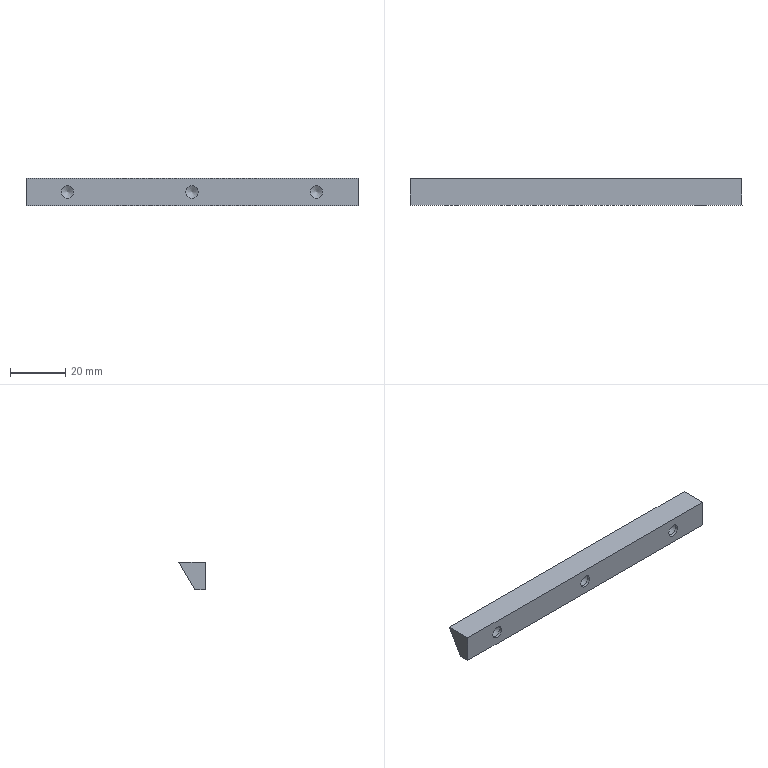Component | NX | SLIDE_GIB_2 | 1 solid | 12 faces | box 120 x 9.5 x 10 mm | volume 7867 mm3 | plane 6 | cone 3 | cylinder 3 | commonest cylinder face diameters 4.5 x3
STEP:
#1=CARTESIAN_POINT('',(0.,0.,0.));
#2=DIRECTION('',(0.,0.,1.));
#3=DIRECTION('',(1.,0.,0.));
#4=AXIS2_PLACEMENT_3D('',#1,#2,#3);
#5=CARTESIAN_POINT('',(-59.8,-54.082,73.));
#6=VERTEX_POINT('',#5);
#7=CARTESIAN_POINT('',(-59.8,-63.582,73.));
#8=VERTEX_POINT('',#7);
#9=CARTESIAN_POINT('',(-59.8,-54.082,73.));
#10=DIRECTION('',(0.,-1.,0.));
#11=VECTOR('',#10,1.);
#12=LINE('',#9,#11);
#13=CARTESIAN_POINT('',(60.2,-54.082,73.));
#14=DIRECTION('',(0.,-0.,-1.));
#15=DIRECTION('',(0.,-1.,0.));
#16=AXIS2_PLACEMENT_3D('',#13,#14,#15);
#17=PLANE('',#16);
#18=CARTESIAN_POINT('',(-0.,120.));
#19=DIRECTION('',(1.,-0.));
#20=VECTOR('',#19,1.);
#21=LINE('',#18,#20);
#22=(GEOMETRIC_REPRESENTATION_CONTEXT(2)PARAMETRIC_REPRESENTATION_CONTEXT()REPRESENTATION_CONTEXT('',''));
#23=DEFINITIONAL_REPRESENTATION('',(#21),#22);
#24=PCURVE('',#17,#23);
#25=CARTESIAN_POINT('',(-59.8,-63.582,68.));
#26=DIRECTION('',(1.,0.,0.));
#27=DIRECTION('',(0.,-1.,0.));
#28=AXIS2_PLACEMENT_3D('',#25,#26,#27);
#29=PLANE('',#28);
#30=CARTESIAN_POINT('',(-9.5,-5.));
#31=DIRECTION('',(1.,-0.));
#32=VECTOR('',#31,1.);
#33=LINE('',#30,#32);
#34=(GEOMETRIC_REPRESENTATION_CONTEXT(2)PARAMETRIC_REPRESENTATION_CONTEXT()REPRESENTATION_CONTEXT('',''));
#35=DEFINITIONAL_REPRESENTATION('',(#33),#34);
#36=PCURVE('',#29,#35);
#37=SURFACE_CURVE('',#12,(#24,#36),.PCURVE_S1.);
#38=EDGE_CURVE('',#6,#8,#37,.T.);
#39=ORIENTED_EDGE('',*,*,#38,.T.);
#40=CARTESIAN_POINT('',(60.2,-63.582,73.));
#41=VERTEX_POINT('',#40);
#42=CARTESIAN_POINT('',(60.2,-63.582,73.));
#43=DIRECTION('',(-1.,-0.,0.));
#44=VECTOR('',#43,1.);
#45=LINE('',#42,#44);
#46=CARTESIAN_POINT('',(9.5,0.));
#47=DIRECTION('',(0.,1.));
#48=VECTOR('',#47,1.);
#49=LINE('',#46,#48);
#50=(GEOMETRIC_REPRESENTATION_CONTEXT(2)PARAMETRIC_REPRESENTATION_CONTEXT()REPRESENTATION_CONTEXT('',''));
#51=DEFINITIONAL_REPRESENTATION('',(#49),#50);
#52=PCURVE('',#17,#51);
#53=CARTESIAN_POINT('',(60.2,-63.582,73.));
#54=DIRECTION('',(-0.,1.,-0.));
#55=DIRECTION('',(-0.,-0.,-1.));
#56=AXIS2_PLACEMENT_3D('',#53,#54,#55);
#57=PLANE('',#56);
#58=CARTESIAN_POINT('',(0.,0.));
#59=DIRECTION('',(0.,1.));
#60=VECTOR('',#59,1.);
#61=LINE('',#58,#60);
#62=(GEOMETRIC_REPRESENTATION_CONTEXT(2)PARAMETRIC_REPRESENTATION_CONTEXT()REPRESENTATION_CONTEXT('',''));
#63=DEFINITIONAL_REPRESENTATION('',(#61),#62);
#64=PCURVE('',#57,#63);
#65=SURFACE_CURVE('',#45,(#52,#64),.PCURVE_S1.);
#66=EDGE_CURVE('',#41,#8,#65,.T.);
#67=ORIENTED_EDGE('',*,*,#66,.F.);
#68=CARTESIAN_POINT('',(60.2,-54.082,73.));
#69=VERTEX_POINT('',#68);
#70=CARTESIAN_POINT('',(60.2,-54.082,73.));
#71=DIRECTION('',(0.,-1.,0.));
#72=VECTOR('',#71,1.);
#73=LINE('',#70,#72);
#74=CARTESIAN_POINT('',(0.,0.));
#75=DIRECTION('',(1.,-0.));
#76=VECTOR('',#75,1.);
#77=LINE('',#74,#76);
#78=(GEOMETRIC_REPRESENTATION_CONTEXT(2)PARAMETRIC_REPRESENTATION_CONTEXT()REPRESENTATION_CONTEXT('',''));
#79=DEFINITIONAL_REPRESENTATION('',(#77),#78);
#80=PCURVE('',#17,#79);
#81=CARTESIAN_POINT('',(60.2,-63.582,68.));
#82=DIRECTION('',(1.,0.,0.));
#83=DIRECTION('',(0.,-1.,0.));
#84=AXIS2_PLACEMENT_3D('',#81,#82,#83);
#85=PLANE('',#84);
#86=CARTESIAN_POINT('',(-9.5,-5.));
#87=DIRECTION('',(1.,-0.));
#88=VECTOR('',#87,1.);
#89=LINE('',#86,#88);
#90=(GEOMETRIC_REPRESENTATION_CONTEXT(2)PARAMETRIC_REPRESENTATION_CONTEXT()REPRESENTATION_CONTEXT('',''));
#91=DEFINITIONAL_REPRESENTATION('',(#89),#90);
#92=PCURVE('',#85,#91);
#93=SURFACE_CURVE('',#73,(#80,#92),.PCURVE_S1.);
#94=EDGE_CURVE('',#69,#41,#93,.T.);
#95=ORIENTED_EDGE('',*,*,#94,.F.);
#96=CARTESIAN_POINT('',(60.2,-54.082,73.));
#97=DIRECTION('',(-1.,-0.,0.));
#98=VECTOR('',#97,1.);
#99=LINE('',#96,#98);
#100=CARTESIAN_POINT('',(0.,0.));
#101=DIRECTION('',(0.,1.));
#102=VECTOR('',#101,1.);
#103=LINE('',#100,#102);
#104=(GEOMETRIC_REPRESENTATION_CONTEXT(2)PARAMETRIC_REPRESENTATION_CONTEXT()REPRESENTATION_CONTEXT('',''));
#105=DEFINITIONAL_REPRESENTATION('',(#103),#104);
#106=PCURVE('',#17,#105);
#107=CARTESIAN_POINT('',(60.2,-59.855,63.));
#108=DIRECTION('',(0.,-0.866,0.5));
#109=DIRECTION('',(-0.,0.5,0.866));
#110=AXIS2_PLACEMENT_3D('',#107,#108,#109);
#111=PLANE('',#110);
#112=CARTESIAN_POINT('',(11.547,-0.));
#113=DIRECTION('',(0.,1.));
#114=VECTOR('',#113,1.);
#115=LINE('',#112,#114);
#116=(GEOMETRIC_REPRESENTATION_CONTEXT(2)PARAMETRIC_REPRESENTATION_CONTEXT()REPRESENTATION_CONTEXT('',''));
#117=DEFINITIONAL_REPRESENTATION('',(#115),#116);
#118=PCURVE('',#111,#117);
#119=SURFACE_CURVE('',#99,(#106,#118),.PCURVE_S1.);
#120=EDGE_CURVE('',#69,#6,#119,.T.);
#121=ORIENTED_EDGE('',*,*,#120,.T.);
#122=EDGE_LOOP('',(#39,#67,#95,#121));
#123=FACE_BOUND('',#122,.T.);
#124=ADVANCED_FACE('',(#123),#17,.F.);
#125=CARTESIAN_POINT('',(-44.8,-63.582,65.75));
#126=VERTEX_POINT('',#125);
#127=CARTESIAN_POINT('',(-44.8,-63.582,68.));
#128=DIRECTION('',(-0.,1.,-0.));
#129=DIRECTION('',(0.,-0.,-1.));
#130=AXIS2_PLACEMENT_3D('',#127,#128,#129);
#131=CIRCLE('',#130,2.25);
#132=CARTESIAN_POINT('',(5.,105.));
#133=DIRECTION('',(1.,-0.));
#134=AXIS2_PLACEMENT_2D('',#132,#133);
#135=CIRCLE('',#134,2.25);
#136=(GEOMETRIC_REPRESENTATION_CONTEXT(2)PARAMETRIC_REPRESENTATION_CONTEXT()REPRESENTATION_CONTEXT('',''));
#137=DEFINITIONAL_REPRESENTATION('',(#135),#136);
#138=PCURVE('',#57,#137);
#139=CARTESIAN_POINT('',(-44.8,-63.582,68.));
#140=DIRECTION('',(-0.,1.,-0.));
#141=DIRECTION('',(0.,-0.,-1.));
#142=AXIS2_PLACEMENT_3D('',#139,#140,#141);
#143=CYLINDRICAL_SURFACE('',#142,2.25);
#144=CARTESIAN_POINT('',(0.,0.));
#145=DIRECTION('',(1.,0.));
#146=VECTOR('',#145,1.);
#147=LINE('',#144,#146);
#148=(GEOMETRIC_REPRESENTATION_CONTEXT(2)PARAMETRIC_REPRESENTATION_CONTEXT()REPRESENTATION_CONTEXT('',''));
#149=DEFINITIONAL_REPRESENTATION('',(#147),#148);
#150=PCURVE('',#143,#149);
#151=SURFACE_CURVE('',#131,(#138,#150),.PCURVE_S1.);
#152=EDGE_CURVE('',#126,#126,#151,.T.);
#153=ORIENTED_EDGE('',*,*,#152,.T.);
#154=EDGE_LOOP('',(#153));
#155=FACE_BOUND('',#154,.T.);
#156=CARTESIAN_POINT('',(0.2,-63.582,65.75));
#157=VERTEX_POINT('',#156);
#158=CARTESIAN_POINT('',(0.2,-63.582,68.));
#159=DIRECTION('',(-0.,1.,-0.));
#160=DIRECTION('',(0.,-0.,-1.));
#161=AXIS2_PLACEMENT_3D('',#158,#159,#160);
#162=CIRCLE('',#161,2.25);
#163=CARTESIAN_POINT('',(5.,60.));
#164=DIRECTION('',(1.,-0.));
#165=AXIS2_PLACEMENT_2D('',#163,#164);
#166=CIRCLE('',#165,2.25);
#167=(GEOMETRIC_REPRESENTATION_CONTEXT(2)PARAMETRIC_REPRESENTATION_CONTEXT()REPRESENTATION_CONTEXT('',''));
#168=DEFINITIONAL_REPRESENTATION('',(#166),#167);
#169=PCURVE('',#57,#168);
#170=CARTESIAN_POINT('',(0.2,-63.582,68.));
#171=DIRECTION('',(-0.,1.,-0.));
#172=DIRECTION('',(0.,-0.,-1.));
#173=AXIS2_PLACEMENT_3D('',#170,#171,#172);
#174=CYLINDRICAL_SURFACE('',#173,2.25);
#175=CARTESIAN_POINT('',(0.,0.));
#176=DIRECTION('',(1.,0.));
#177=VECTOR('',#176,1.);
#178=LINE('',#175,#177);
#179=(GEOMETRIC_REPRESENTATION_CONTEXT(2)PARAMETRIC_REPRESENTATION_CONTEXT()REPRESENTATION_CONTEXT('',''));
#180=DEFINITIONAL_REPRESENTATION('',(#178),#179);
#181=PCURVE('',#174,#180);
#182=SURFACE_CURVE('',#162,(#169,#181),.PCURVE_S1.);
#183=EDGE_CURVE('',#157,#157,#182,.T.);
#184=ORIENTED_EDGE('',*,*,#183,.T.);
#185=EDGE_LOOP('',(#184));
#186=FACE_BOUND('',#185,.T.);
#187=CARTESIAN_POINT('',(45.2,-63.582,65.75));
#188=VERTEX_POINT('',#187);
#189=CARTESIAN_POINT('',(45.2,-63.582,68.));
#190=DIRECTION('',(-0.,1.,-0.));
#191=DIRECTION('',(0.,-0.,-1.));
#192=AXIS2_PLACEMENT_3D('',#189,#190,#191);
#193=CIRCLE('',#192,2.25);
#194=CARTESIAN_POINT('',(5.,15.));
#195=DIRECTION('',(1.,-0.));
#196=AXIS2_PLACEMENT_2D('',#194,#195);
#197=CIRCLE('',#196,2.25);
#198=(GEOMETRIC_REPRESENTATION_CONTEXT(2)PARAMETRIC_REPRESENTATION_CONTEXT()REPRESENTATION_CONTEXT('',''));
#199=DEFINITIONAL_REPRESENTATION('',(#197),#198);
#200=PCURVE('',#57,#199);
#201=CARTESIAN_POINT('',(45.2,-63.582,68.));
#202=DIRECTION('',(-0.,1.,-0.));
#203=DIRECTION('',(0.,-0.,-1.));
#204=AXIS2_PLACEMENT_3D('',#201,#202,#203);
#205=CYLINDRICAL_SURFACE('',#204,2.25);
#206=CARTESIAN_POINT('',(0.,0.));
#207=DIRECTION('',(1.,0.));
#208=VECTOR('',#207,1.);
#209=LINE('',#206,#208);
#210=(GEOMETRIC_REPRESENTATION_CONTEXT(2)PARAMETRIC_REPRESENTATION_CONTEXT()REPRESENTATION_CONTEXT('',''));
#211=DEFINITIONAL_REPRESENTATION('',(#209),#210);
#212=PCURVE('',#205,#211);
#213=SURFACE_CURVE('',#193,(#200,#212),.PCURVE_S1.);
#214=EDGE_CURVE('',#188,#188,#213,.T.);
#215=ORIENTED_EDGE('',*,*,#214,.T.);
#216=EDGE_LOOP('',(#215));
#217=FACE_BOUND('',#216,.T.);
#218=CARTESIAN_POINT('',(-59.8,-63.582,63.));
#219=VERTEX_POINT('',#218);
#220=CARTESIAN_POINT('',(-59.8,-63.582,73.));
#221=DIRECTION('',(0.,-0.,-1.));
#222=VECTOR('',#221,1.);
#223=LINE('',#220,#222);
#224=CARTESIAN_POINT('',(0.,120.));
#225=DIRECTION('',(1.,-0.));
#226=VECTOR('',#225,1.);
#227=LINE('',#224,#226);
#228=(GEOMETRIC_REPRESENTATION_CONTEXT(2)PARAMETRIC_REPRESENTATION_CONTEXT()REPRESENTATION_CONTEXT('',''));
#229=DEFINITIONAL_REPRESENTATION('',(#227),#228);
#230=PCURVE('',#57,#229);
#231=CARTESIAN_POINT('',(0.,-5.));
#232=DIRECTION('',(0.,1.));
#233=VECTOR('',#232,1.);
#234=LINE('',#231,#233);
#235=(GEOMETRIC_REPRESENTATION_CONTEXT(2)PARAMETRIC_REPRESENTATION_CONTEXT()REPRESENTATION_CONTEXT('',''));
#236=DEFINITIONAL_REPRESENTATION('',(#234),#235);
#237=PCURVE('',#29,#236);
#238=SURFACE_CURVE('',#223,(#230,#237),.PCURVE_S1.);
#239=EDGE_CURVE('',#8,#219,#238,.T.);
#240=ORIENTED_EDGE('',*,*,#239,.T.);
#241=CARTESIAN_POINT('',(60.2,-63.582,63.));
#242=VERTEX_POINT('',#241);
#243=CARTESIAN_POINT('',(60.2,-63.582,63.));
#244=DIRECTION('',(-1.,-0.,0.));
#245=VECTOR('',#244,1.);
#246=LINE('',#243,#245);
#247=CARTESIAN_POINT('',(10.,-0.));
#248=DIRECTION('',(0.,1.));
#249=VECTOR('',#248,1.);
#250=LINE('',#247,#249);
#251=(GEOMETRIC_REPRESENTATION_CONTEXT(2)PARAMETRIC_REPRESENTATION_CONTEXT()REPRESENTATION_CONTEXT('',''));
#252=DEFINITIONAL_REPRESENTATION('',(#250),#251);
#253=PCURVE('',#57,#252);
#254=CARTESIAN_POINT('',(60.2,-63.582,63.));
#255=DIRECTION('',(0.,-0.,1.));
#256=DIRECTION('',(-0.,1.,0.));
#257=AXIS2_PLACEMENT_3D('',#254,#255,#256);
#258=PLANE('',#257);
#259=CARTESIAN_POINT('',(0.,0.));
#260=DIRECTION('',(-0.,1.));
#261=VECTOR('',#260,1.);
#262=LINE('',#259,#261);
#263=(GEOMETRIC_REPRESENTATION_CONTEXT(2)PARAMETRIC_REPRESENTATION_CONTEXT()REPRESENTATION_CONTEXT('',''));
#264=DEFINITIONAL_REPRESENTATION('',(#262),#263);
#265=PCURVE('',#258,#264);
#266=SURFACE_CURVE('',#246,(#253,#265),.PCURVE_S1.);
#267=EDGE_CURVE('',#242,#219,#266,.T.);
#268=ORIENTED_EDGE('',*,*,#267,.F.);
#269=CARTESIAN_POINT('',(60.2,-63.582,73.));
#270=DIRECTION('',(0.,-0.,-1.));
#271=VECTOR('',#270,1.);
#272=LINE('',#269,#271);
#273=CARTESIAN_POINT('',(0.,0.));
#274=DIRECTION('',(1.,-0.));
#275=VECTOR('',#274,1.);
#276=LINE('',#273,#275);
#277=(GEOMETRIC_REPRESENTATION_CONTEXT(2)PARAMETRIC_REPRESENTATION_CONTEXT()REPRESENTATION_CONTEXT('',''));
#278=DEFINITIONAL_REPRESENTATION('',(#276),#277);
#279=PCURVE('',#57,#278);
#280=CARTESIAN_POINT('',(0.,-5.));
#281=DIRECTION('',(0.,1.));
#282=VECTOR('',#281,1.);
#283=LINE('',#280,#282);
#284=(GEOMETRIC_REPRESENTATION_CONTEXT(2)PARAMETRIC_REPRESENTATION_CONTEXT()REPRESENTATION_CONTEXT('',''));
#285=DEFINITIONAL_REPRESENTATION('',(#283),#284);
#286=PCURVE('',#85,#285);
#287=SURFACE_CURVE('',#272,(#279,#286),.PCURVE_S1.);
#288=EDGE_CURVE('',#41,#242,#287,.T.);
#289=ORIENTED_EDGE('',*,*,#288,.F.);
#290=ORIENTED_EDGE('',*,*,#66,.T.);
#291=EDGE_LOOP('',(#240,#268,#289,#290));
#292=FACE_BOUND('',#291,.T.);
#293=ADVANCED_FACE('',(#155,#186,#217,#292),#57,.F.);
#294=CARTESIAN_POINT('',(-59.8,-59.855,63.));
#295=VERTEX_POINT('',#294);
#296=CARTESIAN_POINT('',(-59.8,-63.582,63.));
#297=DIRECTION('',(-0.,1.,0.));
#298=VECTOR('',#297,1.);
#299=LINE('',#296,#298);
#300=CARTESIAN_POINT('',(0.,120.));
#301=DIRECTION('',(1.,0.));
#302=VECTOR('',#301,1.);
#303=LINE('',#300,#302);
#304=(GEOMETRIC_REPRESENTATION_CONTEXT(2)PARAMETRIC_REPRESENTATION_CONTEXT()REPRESENTATION_CONTEXT('',''));
#305=DEFINITIONAL_REPRESENTATION('',(#303),#304);
#306=PCURVE('',#258,#305);
#307=CARTESIAN_POINT('',(0.,5.));
#308=DIRECTION('',(-1.,-0.));
#309=VECTOR('',#308,1.);
#310=LINE('',#307,#309);
#311=(GEOMETRIC_REPRESENTATION_CONTEXT(2)PARAMETRIC_REPRESENTATION_CONTEXT()REPRESENTATION_CONTEXT('',''));
#312=DEFINITIONAL_REPRESENTATION('',(#310),#311);
#313=PCURVE('',#29,#312);
#314=SURFACE_CURVE('',#299,(#306,#313),.PCURVE_S1.);
#315=EDGE_CURVE('',#219,#295,#314,.T.);
#316=ORIENTED_EDGE('',*,*,#315,.T.);
#317=CARTESIAN_POINT('',(60.2,-59.855,63.));
#318=VERTEX_POINT('',#317);
#319=CARTESIAN_POINT('',(60.2,-59.855,63.));
#320=DIRECTION('',(-1.,-0.,0.));
#321=VECTOR('',#320,1.);
#322=LINE('',#319,#321);
#323=CARTESIAN_POINT('',(3.726,-0.));
#324=DIRECTION('',(-0.,1.));
#325=VECTOR('',#324,1.);
#326=LINE('',#323,#325);
#327=(GEOMETRIC_REPRESENTATION_CONTEXT(2)PARAMETRIC_REPRESENTATION_CONTEXT()REPRESENTATION_CONTEXT('',''));
#328=DEFINITIONAL_REPRESENTATION('',(#326),#327);
#329=PCURVE('',#258,#328);
#330=CARTESIAN_POINT('',(-0.,0.));
#331=DIRECTION('',(0.,1.));
#332=VECTOR('',#331,1.);
#333=LINE('',#330,#332);
#334=(GEOMETRIC_REPRESENTATION_CONTEXT(2)PARAMETRIC_REPRESENTATION_CONTEXT()REPRESENTATION_CONTEXT('',''));
#335=DEFINITIONAL_REPRESENTATION('',(#333),#334);
#336=PCURVE('',#111,#335);
#337=SURFACE_CURVE('',#322,(#329,#336),.PCURVE_S1.);
#338=EDGE_CURVE('',#318,#295,#337,.T.);
#339=ORIENTED_EDGE('',*,*,#338,.F.);
#340=CARTESIAN_POINT('',(60.2,-63.582,63.));
#341=DIRECTION('',(-0.,1.,0.));
#342=VECTOR('',#341,1.);
#343=LINE('',#340,#342);
#344=CARTESIAN_POINT('',(0.,0.));
#345=DIRECTION('',(1.,0.));
#346=VECTOR('',#345,1.);
#347=LINE('',#344,#346);
#348=(GEOMETRIC_REPRESENTATION_CONTEXT(2)PARAMETRIC_REPRESENTATION_CONTEXT()REPRESENTATION_CONTEXT('',''));
#349=DEFINITIONAL_REPRESENTATION('',(#347),#348);
#350=PCURVE('',#258,#349);
#351=CARTESIAN_POINT('',(0.,5.));
#352=DIRECTION('',(-1.,-0.));
#353=VECTOR('',#352,1.);
#354=LINE('',#351,#353);
#355=(GEOMETRIC_REPRESENTATION_CONTEXT(2)PARAMETRIC_REPRESENTATION_CONTEXT()REPRESENTATION_CONTEXT('',''));
#356=DEFINITIONAL_REPRESENTATION('',(#354),#355);
#357=PCURVE('',#85,#356);
#358=SURFACE_CURVE('',#343,(#350,#357),.PCURVE_S1.);
#359=EDGE_CURVE('',#242,#318,#358,.T.);
#360=ORIENTED_EDGE('',*,*,#359,.F.);
#361=ORIENTED_EDGE('',*,*,#267,.T.);
#362=EDGE_LOOP('',(#316,#339,#360,#361));
#363=FACE_BOUND('',#362,.T.);
#364=ADVANCED_FACE('',(#363),#258,.F.);
#365=CARTESIAN_POINT('',(-59.8,-59.855,63.));
#366=DIRECTION('',(-0.,0.5,0.866));
#367=VECTOR('',#366,1.);
#368=LINE('',#365,#367);
#369=CARTESIAN_POINT('',(0.,120.));
#370=DIRECTION('',(1.,-0.));
#371=VECTOR('',#370,1.);
#372=LINE('',#369,#371);
#373=(GEOMETRIC_REPRESENTATION_CONTEXT(2)PARAMETRIC_REPRESENTATION_CONTEXT()REPRESENTATION_CONTEXT('',''));
#374=DEFINITIONAL_REPRESENTATION('',(#372),#373);
#375=PCURVE('',#111,#374);
#376=CARTESIAN_POINT('',(-3.726,5.));
#377=DIRECTION('',(-0.5,-0.866));
#378=VECTOR('',#377,1.);
#379=LINE('',#376,#378);
#380=(GEOMETRIC_REPRESENTATION_CONTEXT(2)PARAMETRIC_REPRESENTATION_CONTEXT()REPRESENTATION_CONTEXT('',''));
#381=DEFINITIONAL_REPRESENTATION('',(#379),#380);
#382=PCURVE('',#29,#381);
#383=SURFACE_CURVE('',#368,(#375,#382),.PCURVE_S1.);
#384=EDGE_CURVE('',#295,#6,#383,.T.);
#385=ORIENTED_EDGE('',*,*,#384,.T.);
#386=ORIENTED_EDGE('',*,*,#120,.F.);
#387=CARTESIAN_POINT('',(60.2,-59.855,63.));
#388=DIRECTION('',(-0.,0.5,0.866));
#389=VECTOR('',#388,1.);
#390=LINE('',#387,#389);
#391=CARTESIAN_POINT('',(0.,0.));
#392=DIRECTION('',(1.,-0.));
#393=VECTOR('',#392,1.);
#394=LINE('',#391,#393);
#395=(GEOMETRIC_REPRESENTATION_CONTEXT(2)PARAMETRIC_REPRESENTATION_CONTEXT()REPRESENTATION_CONTEXT('',''));
#396=DEFINITIONAL_REPRESENTATION('',(#394),#395);
#397=PCURVE('',#111,#396);
#398=CARTESIAN_POINT('',(-3.726,5.));
#399=DIRECTION('',(-0.5,-0.866));
#400=VECTOR('',#399,1.);
#401=LINE('',#398,#400);
#402=(GEOMETRIC_REPRESENTATION_CONTEXT(2)PARAMETRIC_REPRESENTATION_CONTEXT()REPRESENTATION_CONTEXT('',''));
#403=DEFINITIONAL_REPRESENTATION('',(#401),#402);
#404=PCURVE('',#85,#403);
#405=SURFACE_CURVE('',#390,(#397,#404),.PCURVE_S1.);
#406=EDGE_CURVE('',#318,#69,#405,.T.);
#407=ORIENTED_EDGE('',*,*,#406,.F.);
#408=ORIENTED_EDGE('',*,*,#338,.T.);
#409=EDGE_LOOP('',(#385,#386,#407,#408));
#410=FACE_BOUND('',#409,.T.);
#411=ADVANCED_FACE('',(#410),#111,.F.);
#412=ORIENTED_EDGE('',*,*,#94,.T.);
#413=ORIENTED_EDGE('',*,*,#288,.T.);
#414=ORIENTED_EDGE('',*,*,#359,.T.);
#415=ORIENTED_EDGE('',*,*,#406,.T.);
#416=EDGE_LOOP('',(#412,#413,#414,#415));
#417=FACE_BOUND('',#416,.T.);
#418=ADVANCED_FACE('',(#417),#85,.T.);
#419=ORIENTED_EDGE('',*,*,#38,.F.);
#420=ORIENTED_EDGE('',*,*,#384,.F.);
#421=ORIENTED_EDGE('',*,*,#315,.F.);
#422=ORIENTED_EDGE('',*,*,#239,.F.);
#423=EDGE_LOOP('',(#419,#420,#421,#422));
#424=FACE_BOUND('',#423,.T.);
#425=ADVANCED_FACE('',(#424),#29,.F.);
#426=CARTESIAN_POINT('',(45.2,-62.582,70.25));
#427=VERTEX_POINT('',#426);
#428=CARTESIAN_POINT('',(45.2,-62.582,65.75));
#429=VERTEX_POINT('',#428);
#430=CARTESIAN_POINT('',(45.2,-62.582,68.));
#431=DIRECTION('',(0.,-1.,0.));
#432=DIRECTION('',(0.,-0.,-1.));
#433=AXIS2_PLACEMENT_3D('',#430,#431,#432);
#434=CIRCLE('',#433,2.25);
#435=CARTESIAN_POINT('',(45.2,-62.582,68.));
#436=DIRECTION('',(0.,-1.,0.));
#437=DIRECTION('',(0.,0.,1.));
#438=AXIS2_PLACEMENT_3D('',#435,#436,#437);
#439=CONICAL_SURFACE('',#438,2.25,1.03);
#440=CARTESIAN_POINT('',(-3.142,-0.));
#441=DIRECTION('',(1.,0.));
#442=VECTOR('',#441,1.);
#443=LINE('',#440,#442);
#444=(GEOMETRIC_REPRESENTATION_CONTEXT(2)PARAMETRIC_REPRESENTATION_CONTEXT()REPRESENTATION_CONTEXT('',''));
#445=DEFINITIONAL_REPRESENTATION('',(#443),#444);
#446=PCURVE('',#439,#445);
#447=CARTESIAN_POINT('',(6.283,1.));
#448=DIRECTION('',(-1.,0.));
#449=VECTOR('',#448,1.);
#450=LINE('',#447,#449);
#451=(GEOMETRIC_REPRESENTATION_CONTEXT(2)PARAMETRIC_REPRESENTATION_CONTEXT()REPRESENTATION_CONTEXT('',''));
#452=DEFINITIONAL_REPRESENTATION('',(#450),#451);
#453=PCURVE('',#205,#452);
#454=SURFACE_CURVE('',#434,(#446,#453),.PCURVE_S1.);
#455=EDGE_CURVE('',#427,#429,#454,.T.);
#456=ORIENTED_EDGE('',*,*,#455,.F.);
#457=CARTESIAN_POINT('',(45.2,-61.23,68.));
#458=VERTEX_POINT('',#457);
#459=CARTESIAN_POINT('',(45.2,-61.23,68.));
#460=CARTESIAN_POINT('',(45.2,-62.582,70.25));
#461=B_SPLINE_CURVE_WITH_KNOTS('',1,(#459,#460),.UNSPECIFIED.,.F.,.F.,(2,2),(-2.625,-0.),.PIECEWISE_BEZIER_KNOTS.);
#462=CARTESIAN_POINT('',(0.,0.));
#463=DIRECTION('',(0.,1.));
#464=VECTOR('',#463,1.);
#465=LINE('',#462,#464);
#466=(GEOMETRIC_REPRESENTATION_CONTEXT(2)PARAMETRIC_REPRESENTATION_CONTEXT()REPRESENTATION_CONTEXT('',''));
#467=DEFINITIONAL_REPRESENTATION('',(#465),#466);
#468=PCURVE('',#439,#467);
#469=CARTESIAN_POINT('',(6.283,0.));
#470=DIRECTION('',(0.,1.));
#471=VECTOR('',#470,1.);
#472=LINE('',#469,#471);
#473=(GEOMETRIC_REPRESENTATION_CONTEXT(2)PARAMETRIC_REPRESENTATION_CONTEXT()REPRESENTATION_CONTEXT('',''));
#474=DEFINITIONAL_REPRESENTATION('',(#472),#473);
#475=PCURVE('',#439,#474);
#476=SEAM_CURVE('',#461,(#468,#475),.PCURVE_S1.);
#477=EDGE_CURVE('',#458,#427,#476,.T.);
#478=ORIENTED_EDGE('',*,*,#477,.F.);
#479=ORIENTED_EDGE('',*,*,#477,.T.);
#480=CARTESIAN_POINT('',(45.2,-62.582,68.));
#481=DIRECTION('',(0.,-1.,0.));
#482=DIRECTION('',(0.,-0.,-1.));
#483=AXIS2_PLACEMENT_3D('',#480,#481,#482);
#484=CIRCLE('',#483,2.25);
#485=CARTESIAN_POINT('',(3.142,-0.));
#486=DIRECTION('',(1.,0.));
#487=VECTOR('',#486,1.);
#488=LINE('',#485,#487);
#489=(GEOMETRIC_REPRESENTATION_CONTEXT(2)PARAMETRIC_REPRESENTATION_CONTEXT()REPRESENTATION_CONTEXT('',''));
#490=DEFINITIONAL_REPRESENTATION('',(#488),#489);
#491=PCURVE('',#439,#490);
#492=CARTESIAN_POINT('',(6.283,1.));
#493=DIRECTION('',(-1.,-0.));
#494=VECTOR('',#493,1.);
#495=LINE('',#492,#494);
#496=(GEOMETRIC_REPRESENTATION_CONTEXT(2)PARAMETRIC_REPRESENTATION_CONTEXT()REPRESENTATION_CONTEXT('',''));
#497=DEFINITIONAL_REPRESENTATION('',(#495),#496);
#498=PCURVE('',#205,#497);
#499=SURFACE_CURVE('',#484,(#491,#498),.PCURVE_S1.);
#500=EDGE_CURVE('',#429,#427,#499,.T.);
#501=ORIENTED_EDGE('',*,*,#500,.F.);
#502=EDGE_LOOP('',(#456,#478,#479,#501));
#503=FACE_BOUND('',#502,.F.);
#504=ADVANCED_FACE('',(#503),#439,.F.);
#505=ORIENTED_EDGE('',*,*,#455,.T.);
#506=CARTESIAN_POINT('',(45.2,-63.582,65.75));
#507=CARTESIAN_POINT('',(45.2,-62.582,65.75));
#508=B_SPLINE_CURVE_WITH_KNOTS('',1,(#506,#507),.UNSPECIFIED.,.F.,.F.,(2,2),(0.,1.),.PIECEWISE_BEZIER_KNOTS.);
#509=CARTESIAN_POINT('',(0.,0.));
#510=DIRECTION('',(0.,1.));
#511=VECTOR('',#510,1.);
#512=LINE('',#509,#511);
#513=(GEOMETRIC_REPRESENTATION_CONTEXT(2)PARAMETRIC_REPRESENTATION_CONTEXT()REPRESENTATION_CONTEXT('',''));
#514=DEFINITIONAL_REPRESENTATION('',(#512),#513);
#515=PCURVE('',#205,#514);
#516=CARTESIAN_POINT('',(6.283,0.));
#517=DIRECTION('',(0.,1.));
#518=VECTOR('',#517,1.);
#519=LINE('',#516,#518);
#520=(GEOMETRIC_REPRESENTATION_CONTEXT(2)PARAMETRIC_REPRESENTATION_CONTEXT()REPRESENTATION_CONTEXT('',''));
#521=DEFINITIONAL_REPRESENTATION('',(#519),#520);
#522=PCURVE('',#205,#521);
#523=SEAM_CURVE('',#508,(#515,#522),.PCURVE_S1.);
#524=EDGE_CURVE('',#188,#429,#523,.T.);
#525=ORIENTED_EDGE('',*,*,#524,.F.);
#526=ORIENTED_EDGE('',*,*,#214,.T.);
#527=ORIENTED_EDGE('',*,*,#524,.T.);
#528=ORIENTED_EDGE('',*,*,#500,.T.);
#529=EDGE_LOOP('',(#505,#525,#526,#527,#528));
#530=FACE_BOUND('',#529,.F.);
#531=ADVANCED_FACE('',(#530),#205,.F.);
#532=CARTESIAN_POINT('',(0.2,-62.582,70.25));
#533=VERTEX_POINT('',#532);
#534=CARTESIAN_POINT('',(0.2,-62.582,65.75));
#535=VERTEX_POINT('',#534);
#536=CARTESIAN_POINT('',(0.2,-62.582,68.));
#537=DIRECTION('',(0.,-1.,0.));
#538=DIRECTION('',(0.,-0.,-1.));
#539=AXIS2_PLACEMENT_3D('',#536,#537,#538);
#540=CIRCLE('',#539,2.25);
#541=CARTESIAN_POINT('',(0.2,-62.582,68.));
#542=DIRECTION('',(0.,-1.,0.));
#543=DIRECTION('',(0.,0.,1.));
#544=AXIS2_PLACEMENT_3D('',#541,#542,#543);
#545=CONICAL_SURFACE('',#544,2.25,1.03);
#546=CARTESIAN_POINT('',(-3.142,-0.));
#547=DIRECTION('',(1.,0.));
#548=VECTOR('',#547,1.);
#549=LINE('',#546,#548);
#550=(GEOMETRIC_REPRESENTATION_CONTEXT(2)PARAMETRIC_REPRESENTATION_CONTEXT()REPRESENTATION_CONTEXT('',''));
#551=DEFINITIONAL_REPRESENTATION('',(#549),#550);
#552=PCURVE('',#545,#551);
#553=CARTESIAN_POINT('',(6.283,1.));
#554=DIRECTION('',(-1.,0.));
#555=VECTOR('',#554,1.);
#556=LINE('',#553,#555);
#557=(GEOMETRIC_REPRESENTATION_CONTEXT(2)PARAMETRIC_REPRESENTATION_CONTEXT()REPRESENTATION_CONTEXT('',''));
#558=DEFINITIONAL_REPRESENTATION('',(#556),#557);
#559=PCURVE('',#174,#558);
#560=SURFACE_CURVE('',#540,(#552,#559),.PCURVE_S1.);
#561=EDGE_CURVE('',#533,#535,#560,.T.);
#562=ORIENTED_EDGE('',*,*,#561,.F.);
#563=CARTESIAN_POINT('',(0.2,-61.23,68.));
#564=VERTEX_POINT('',#563);
#565=CARTESIAN_POINT('',(0.2,-61.23,68.));
#566=CARTESIAN_POINT('',(0.2,-62.582,70.25));
#567=B_SPLINE_CURVE_WITH_KNOTS('',1,(#565,#566),.UNSPECIFIED.,.F.,.F.,(2,2),(-2.625,-0.),.PIECEWISE_BEZIER_KNOTS.);
#568=CARTESIAN_POINT('',(0.,0.));
#569=DIRECTION('',(0.,1.));
#570=VECTOR('',#569,1.);
#571=LINE('',#568,#570);
#572=(GEOMETRIC_REPRESENTATION_CONTEXT(2)PARAMETRIC_REPRESENTATION_CONTEXT()REPRESENTATION_CONTEXT('',''));
#573=DEFINITIONAL_REPRESENTATION('',(#571),#572);
#574=PCURVE('',#545,#573);
#575=CARTESIAN_POINT('',(6.283,0.));
#576=DIRECTION('',(0.,1.));
#577=VECTOR('',#576,1.);
#578=LINE('',#575,#577);
#579=(GEOMETRIC_REPRESENTATION_CONTEXT(2)PARAMETRIC_REPRESENTATION_CONTEXT()REPRESENTATION_CONTEXT('',''));
#580=DEFINITIONAL_REPRESENTATION('',(#578),#579);
#581=PCURVE('',#545,#580);
#582=SEAM_CURVE('',#567,(#574,#581),.PCURVE_S1.);
#583=EDGE_CURVE('',#564,#533,#582,.T.);
#584=ORIENTED_EDGE('',*,*,#583,.F.);
#585=ORIENTED_EDGE('',*,*,#583,.T.);
#586=CARTESIAN_POINT('',(0.2,-62.582,68.));
#587=DIRECTION('',(0.,-1.,0.));
#588=DIRECTION('',(0.,-0.,-1.));
#589=AXIS2_PLACEMENT_3D('',#586,#587,#588);
#590=CIRCLE('',#589,2.25);
#591=CARTESIAN_POINT('',(3.142,-0.));
#592=DIRECTION('',(1.,0.));
#593=VECTOR('',#592,1.);
#594=LINE('',#591,#593);
#595=(GEOMETRIC_REPRESENTATION_CONTEXT(2)PARAMETRIC_REPRESENTATION_CONTEXT()REPRESENTATION_CONTEXT('',''));
#596=DEFINITIONAL_REPRESENTATION('',(#594),#595);
#597=PCURVE('',#545,#596);
#598=CARTESIAN_POINT('',(6.283,1.));
#599=DIRECTION('',(-1.,-0.));
#600=VECTOR('',#599,1.);
#601=LINE('',#598,#600);
#602=(GEOMETRIC_REPRESENTATION_CONTEXT(2)PARAMETRIC_REPRESENTATION_CONTEXT()REPRESENTATION_CONTEXT('',''));
#603=DEFINITIONAL_REPRESENTATION('',(#601),#602);
#604=PCURVE('',#174,#603);
#605=SURFACE_CURVE('',#590,(#597,#604),.PCURVE_S1.);
#606=EDGE_CURVE('',#535,#533,#605,.T.);
#607=ORIENTED_EDGE('',*,*,#606,.F.);
#608=EDGE_LOOP('',(#562,#584,#585,#607));
#609=FACE_BOUND('',#608,.F.);
#610=ADVANCED_FACE('',(#609),#545,.F.);
#611=ORIENTED_EDGE('',*,*,#561,.T.);
#612=CARTESIAN_POINT('',(0.2,-63.582,65.75));
#613=CARTESIAN_POINT('',(0.2,-62.582,65.75));
#614=B_SPLINE_CURVE_WITH_KNOTS('',1,(#612,#613),.UNSPECIFIED.,.F.,.F.,(2,2),(0.,1.),.PIECEWISE_BEZIER_KNOTS.);
#615=CARTESIAN_POINT('',(0.,0.));
#616=DIRECTION('',(0.,1.));
#617=VECTOR('',#616,1.);
#618=LINE('',#615,#617);
#619=(GEOMETRIC_REPRESENTATION_CONTEXT(2)PARAMETRIC_REPRESENTATION_CONTEXT()REPRESENTATION_CONTEXT('',''));
#620=DEFINITIONAL_REPRESENTATION('',(#618),#619);
#621=PCURVE('',#174,#620);
#622=CARTESIAN_POINT('',(6.283,0.));
#623=DIRECTION('',(0.,1.));
#624=VECTOR('',#623,1.);
#625=LINE('',#622,#624);
#626=(GEOMETRIC_REPRESENTATION_CONTEXT(2)PARAMETRIC_REPRESENTATION_CONTEXT()REPRESENTATION_CONTEXT('',''));
#627=DEFINITIONAL_REPRESENTATION('',(#625),#626);
#628=PCURVE('',#174,#627);
#629=SEAM_CURVE('',#614,(#621,#628),.PCURVE_S1.);
#630=EDGE_CURVE('',#157,#535,#629,.T.);
#631=ORIENTED_EDGE('',*,*,#630,.F.);
#632=ORIENTED_EDGE('',*,*,#183,.T.);
#633=ORIENTED_EDGE('',*,*,#630,.T.);
#634=ORIENTED_EDGE('',*,*,#606,.T.);
#635=EDGE_LOOP('',(#611,#631,#632,#633,#634));
#636=FACE_BOUND('',#635,.F.);
#637=ADVANCED_FACE('',(#636),#174,.F.);
#638=CARTESIAN_POINT('',(-44.8,-62.582,70.25));
#639=VERTEX_POINT('',#638);
#640=CARTESIAN_POINT('',(-44.8,-62.582,65.75));
#641=VERTEX_POINT('',#640);
#642=CARTESIAN_POINT('',(-44.8,-62.582,68.));
#643=DIRECTION('',(0.,-1.,0.));
#644=DIRECTION('',(0.,-0.,-1.));
#645=AXIS2_PLACEMENT_3D('',#642,#643,#644);
#646=CIRCLE('',#645,2.25);
#647=CARTESIAN_POINT('',(-44.8,-62.582,68.));
#648=DIRECTION('',(0.,-1.,0.));
#649=DIRECTION('',(0.,0.,1.));
#650=AXIS2_PLACEMENT_3D('',#647,#648,#649);
#651=CONICAL_SURFACE('',#650,2.25,1.03);
#652=CARTESIAN_POINT('',(-3.142,-0.));
#653=DIRECTION('',(1.,0.));
#654=VECTOR('',#653,1.);
#655=LINE('',#652,#654);
#656=(GEOMETRIC_REPRESENTATION_CONTEXT(2)PARAMETRIC_REPRESENTATION_CONTEXT()REPRESENTATION_CONTEXT('',''));
#657=DEFINITIONAL_REPRESENTATION('',(#655),#656);
#658=PCURVE('',#651,#657);
#659=CARTESIAN_POINT('',(6.283,1.));
#660=DIRECTION('',(-1.,0.));
#661=VECTOR('',#660,1.);
#662=LINE('',#659,#661);
#663=(GEOMETRIC_REPRESENTATION_CONTEXT(2)PARAMETRIC_REPRESENTATION_CONTEXT()REPRESENTATION_CONTEXT('',''));
#664=DEFINITIONAL_REPRESENTATION('',(#662),#663);
#665=PCURVE('',#143,#664);
#666=SURFACE_CURVE('',#646,(#658,#665),.PCURVE_S1.);
#667=EDGE_CURVE('',#639,#641,#666,.T.);
#668=ORIENTED_EDGE('',*,*,#667,.F.);
#669=CARTESIAN_POINT('',(-44.8,-61.23,68.));
#670=VERTEX_POINT('',#669);
#671=CARTESIAN_POINT('',(-44.8,-61.23,68.));
#672=CARTESIAN_POINT('',(-44.8,-62.582,70.25));
#673=B_SPLINE_CURVE_WITH_KNOTS('',1,(#671,#672),.UNSPECIFIED.,.F.,.F.,(2,2),(-2.625,-0.),.PIECEWISE_BEZIER_KNOTS.);
#674=CARTESIAN_POINT('',(0.,0.));
#675=DIRECTION('',(0.,1.));
#676=VECTOR('',#675,1.);
#677=LINE('',#674,#676);
#678=(GEOMETRIC_REPRESENTATION_CONTEXT(2)PARAMETRIC_REPRESENTATION_CONTEXT()REPRESENTATION_CONTEXT('',''));
#679=DEFINITIONAL_REPRESENTATION('',(#677),#678);
#680=PCURVE('',#651,#679);
#681=CARTESIAN_POINT('',(6.283,0.));
#682=DIRECTION('',(0.,1.));
#683=VECTOR('',#682,1.);
#684=LINE('',#681,#683);
#685=(GEOMETRIC_REPRESENTATION_CONTEXT(2)PARAMETRIC_REPRESENTATION_CONTEXT()REPRESENTATION_CONTEXT('',''));
#686=DEFINITIONAL_REPRESENTATION('',(#684),#685);
#687=PCURVE('',#651,#686);
#688=SEAM_CURVE('',#673,(#680,#687),.PCURVE_S1.);
#689=EDGE_CURVE('',#670,#639,#688,.T.);
#690=ORIENTED_EDGE('',*,*,#689,.F.);
#691=ORIENTED_EDGE('',*,*,#689,.T.);
#692=CARTESIAN_POINT('',(-44.8,-62.582,68.));
#693=DIRECTION('',(0.,-1.,0.));
#694=DIRECTION('',(0.,-0.,-1.));
#695=AXIS2_PLACEMENT_3D('',#692,#693,#694);
#696=CIRCLE('',#695,2.25);
#697=CARTESIAN_POINT('',(3.142,-0.));
#698=DIRECTION('',(1.,0.));
#699=VECTOR('',#698,1.);
#700=LINE('',#697,#699);
#701=(GEOMETRIC_REPRESENTATION_CONTEXT(2)PARAMETRIC_REPRESENTATION_CONTEXT()REPRESENTATION_CONTEXT('',''));
#702=DEFINITIONAL_REPRESENTATION('',(#700),#701);
#703=PCURVE('',#651,#702);
#704=CARTESIAN_POINT('',(6.283,1.));
#705=DIRECTION('',(-1.,-0.));
#706=VECTOR('',#705,1.);
#707=LINE('',#704,#706);
#708=(GEOMETRIC_REPRESENTATION_CONTEXT(2)PARAMETRIC_REPRESENTATION_CONTEXT()REPRESENTATION_CONTEXT('',''));
#709=DEFINITIONAL_REPRESENTATION('',(#707),#708);
#710=PCURVE('',#143,#709);
#711=SURFACE_CURVE('',#696,(#703,#710),.PCURVE_S1.);
#712=EDGE_CURVE('',#641,#639,#711,.T.);
#713=ORIENTED_EDGE('',*,*,#712,.F.);
#714=EDGE_LOOP('',(#668,#690,#691,#713));
#715=FACE_BOUND('',#714,.F.);
#716=ADVANCED_FACE('',(#715),#651,.F.);
#717=ORIENTED_EDGE('',*,*,#667,.T.);
#718=CARTESIAN_POINT('',(-44.8,-63.582,65.75));
#719=CARTESIAN_POINT('',(-44.8,-62.582,65.75));
#720=B_SPLINE_CURVE_WITH_KNOTS('',1,(#718,#719),.UNSPECIFIED.,.F.,.F.,(2,2),(0.,1.),.PIECEWISE_BEZIER_KNOTS.);
#721=CARTESIAN_POINT('',(0.,0.));
#722=DIRECTION('',(0.,1.));
#723=VECTOR('',#722,1.);
#724=LINE('',#721,#723);
#725=(GEOMETRIC_REPRESENTATION_CONTEXT(2)PARAMETRIC_REPRESENTATION_CONTEXT()REPRESENTATION_CONTEXT('',''));
#726=DEFINITIONAL_REPRESENTATION('',(#724),#725);
#727=PCURVE('',#143,#726);
#728=CARTESIAN_POINT('',(6.283,0.));
#729=DIRECTION('',(0.,1.));
#730=VECTOR('',#729,1.);
#731=LINE('',#728,#730);
#732=(GEOMETRIC_REPRESENTATION_CONTEXT(2)PARAMETRIC_REPRESENTATION_CONTEXT()REPRESENTATION_CONTEXT('',''));
#733=DEFINITIONAL_REPRESENTATION('',(#731),#732);
#734=PCURVE('',#143,#733);
#735=SEAM_CURVE('',#720,(#727,#734),.PCURVE_S1.);
#736=EDGE_CURVE('',#126,#641,#735,.T.);
#737=ORIENTED_EDGE('',*,*,#736,.F.);
#738=ORIENTED_EDGE('',*,*,#152,.T.);
#739=ORIENTED_EDGE('',*,*,#736,.T.);
#740=ORIENTED_EDGE('',*,*,#712,.T.);
#741=EDGE_LOOP('',(#717,#737,#738,#739,#740));
#742=FACE_BOUND('',#741,.F.);
#743=ADVANCED_FACE('',(#742),#143,.F.);
#744=CLOSED_SHELL('',(#124,#293,#364,#411,#418,#425,#504,#531,#610,#637,#716,#743));
#745=MANIFOLD_SOLID_BREP('',#744);
#746=(LENGTH_UNIT()NAMED_UNIT(*)SI_UNIT(.MILLI.,.METRE.));
#747=UNCERTAINTY_MEASURE_WITH_UNIT(LENGTH_MEASURE(0.000005),#746,'','');
#748=(NAMED_UNIT(*)PLANE_ANGLE_UNIT()SI_UNIT($,.RADIAN.));
#749=(NAMED_UNIT(*)SI_UNIT($,.STERADIAN.)SOLID_ANGLE_UNIT());
#750=(GEOMETRIC_REPRESENTATION_CONTEXT(3)GLOBAL_UNCERTAINTY_ASSIGNED_CONTEXT((#747))GLOBAL_UNIT_ASSIGNED_CONTEXT((#746,#748,#749))REPRESENTATION_CONTEXT('',''));
#751=ADVANCED_BREP_SHAPE_REPRESENTATION('',(#4,#745),#750);